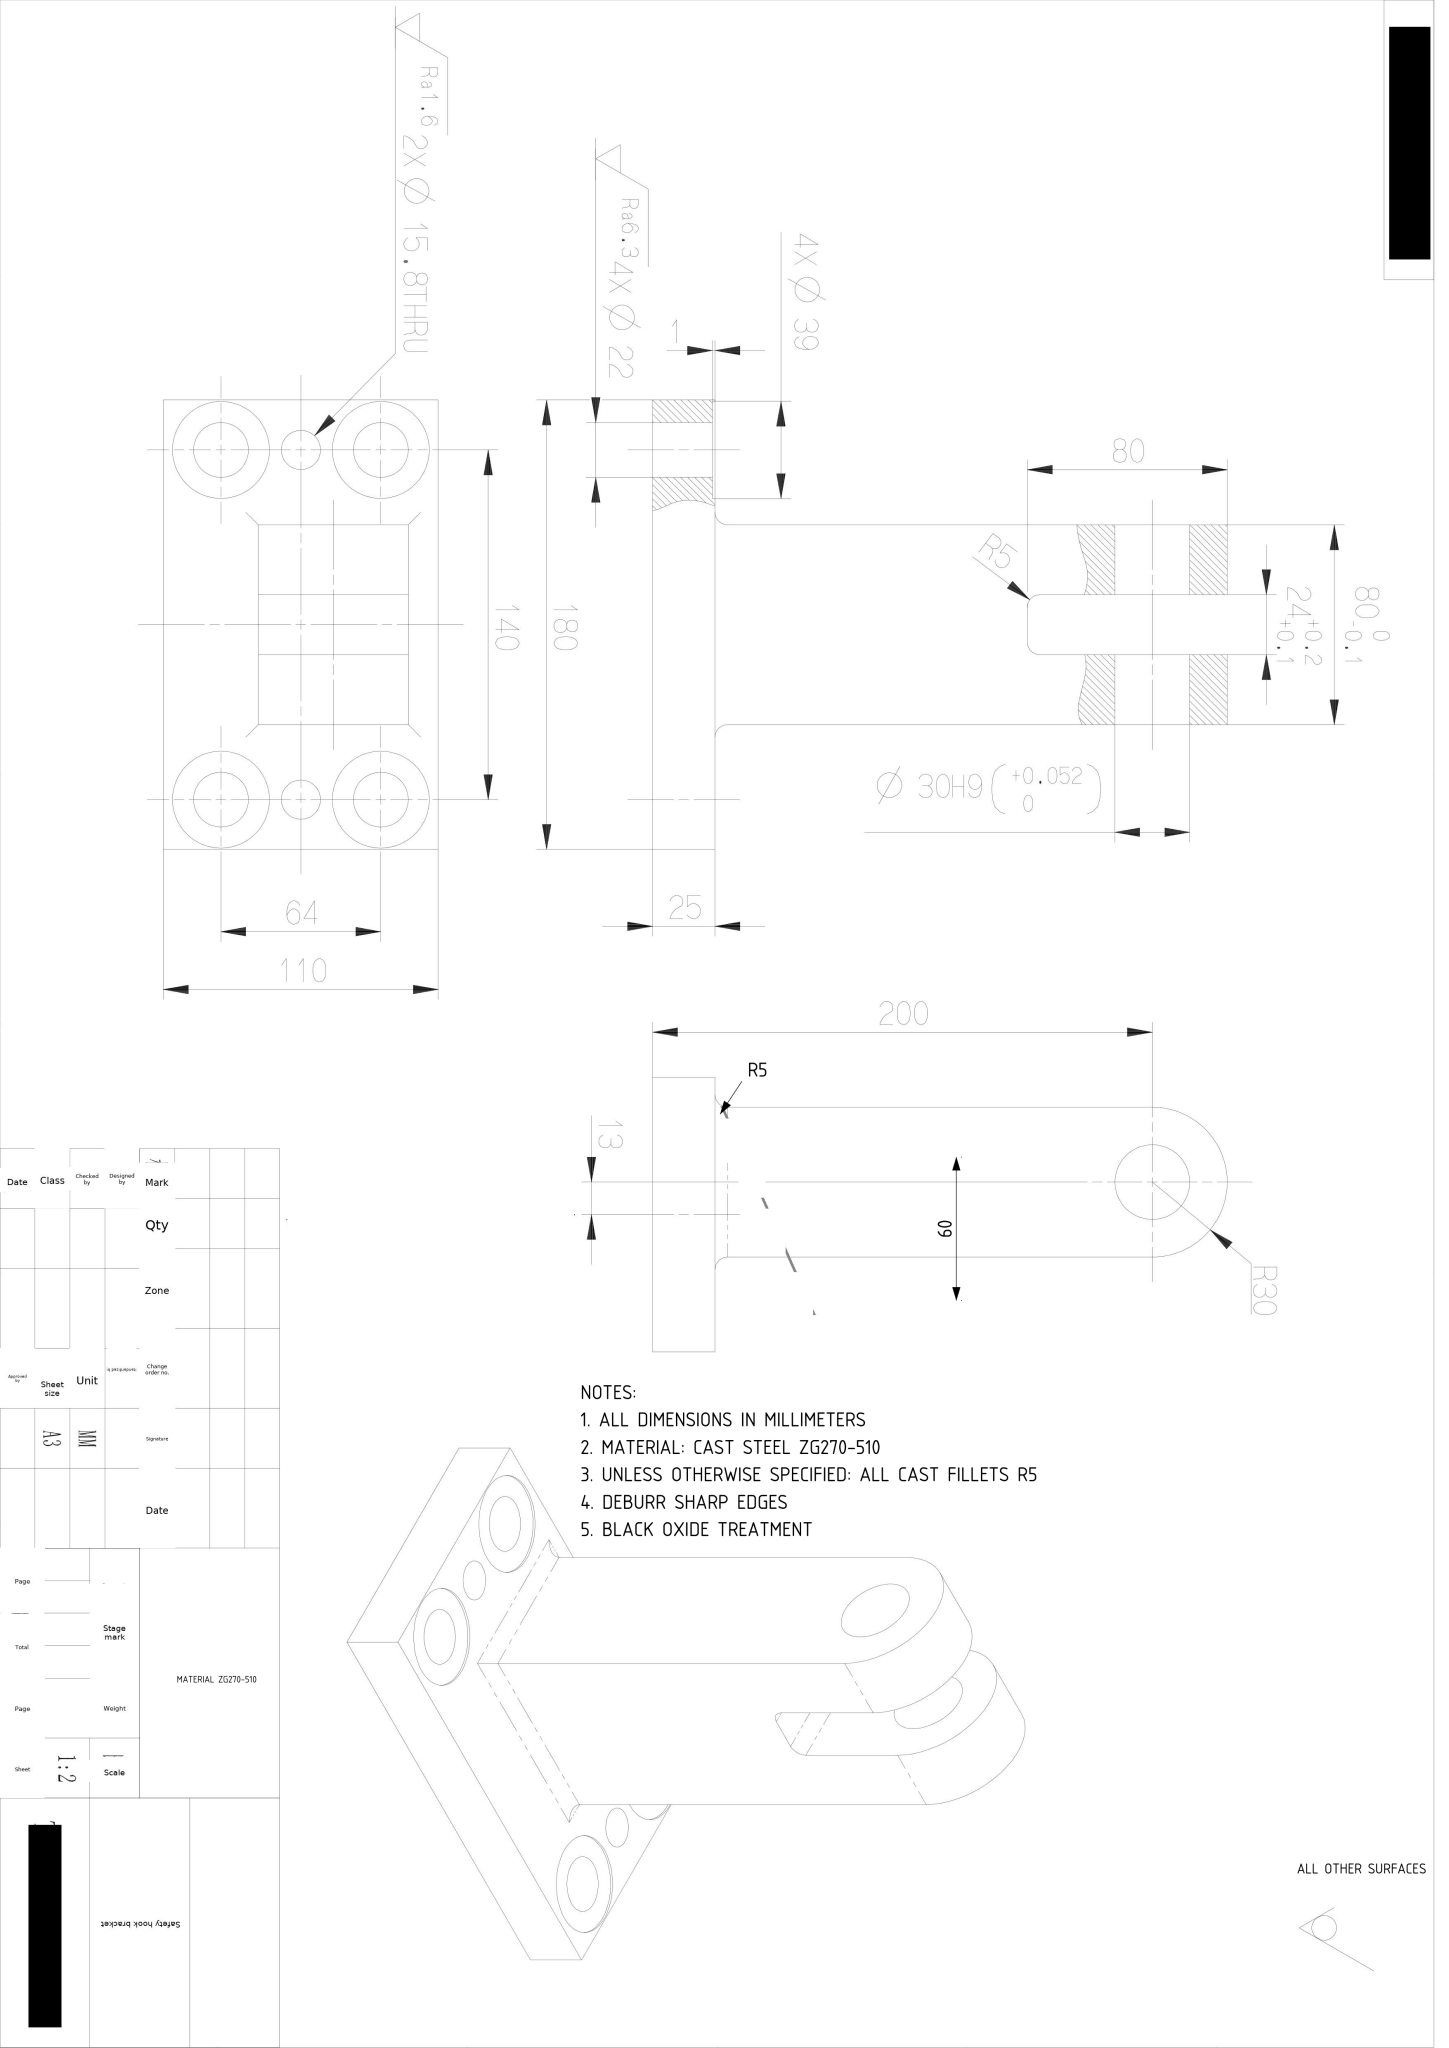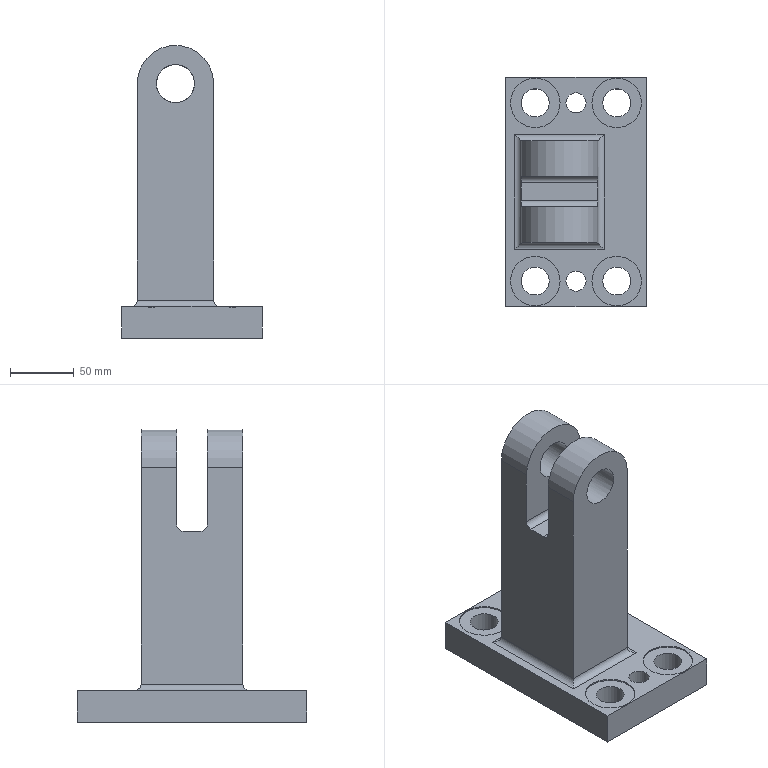Part | NX | mm | 1 solid | 37 faces | box 110 x 180 x 230 mm | volume 1253704 mm3 | cylinder 20 | plane 17 | commonest cylinder face diameters 10 x6 22 x4 39 x4 60 x2 30 x2 15.8 x2
STEP:
#1=CARTESIAN_POINT('',(0.,0.,0.));
#2=DIRECTION('',(0.,0.,1.));
#3=DIRECTION('',(1.,0.,0.));
#4=AXIS2_PLACEMENT_3D('',#1,#2,#3);
#5=(LENGTH_UNIT()NAMED_UNIT(*)SI_UNIT(.MILLI.,.METRE.));
#6=UNCERTAINTY_MEASURE_WITH_UNIT(LENGTH_MEASURE(0.00002),#5,'','');
#7=(NAMED_UNIT(*)PLANE_ANGLE_UNIT()SI_UNIT($,.RADIAN.));
#8=PLANE_ANGLE_MEASURE_WITH_UNIT(PLANE_ANGLE_MEASURE(0.01745),#7);
#9=DIMENSIONAL_EXPONENTS(0.,0.,0.,0.,0.,0.,0.);
#10=(CONVERSION_BASED_UNIT('',#8)NAMED_UNIT(#9)PLANE_ANGLE_UNIT());
#11=(NAMED_UNIT(*)SI_UNIT($,.STERADIAN.)SOLID_ANGLE_UNIT());
#12=(GEOMETRIC_REPRESENTATION_CONTEXT(3)GLOBAL_UNCERTAINTY_ASSIGNED_CONTEXT((#6))GLOBAL_UNIT_ASSIGNED_CONTEXT((#5,#10,#11))REPRESENTATION_CONTEXT('',''));
#13=SHAPE_REPRESENTATION('',(#4),#12);
#14=CARTESIAN_POINT('',(17.,-40.,200.));
#15=VERTEX_POINT('',#14);
#16=CARTESIAN_POINT('',(17.,-40.,30.));
#17=VERTEX_POINT('',#16);
#18=CARTESIAN_POINT('',(17.,-40.,230.));
#19=DIRECTION('',(0.,0.,-1.));
#20=VECTOR('',#19,1.);
#21=LINE('',#18,#20);
#22=EDGE_CURVE('',#15,#17,#21,.T.);
#23=ORIENTED_EDGE('',*,*,#22,.T.);
#24=CARTESIAN_POINT('',(17.,40.,30.));
#25=VERTEX_POINT('',#24);
#26=CARTESIAN_POINT('',(17.,-40.,30.));
#27=DIRECTION('',(-0.,1.,0.));
#28=VECTOR('',#27,1.);
#29=LINE('',#26,#28);
#30=EDGE_CURVE('',#17,#25,#29,.T.);
#31=ORIENTED_EDGE('',*,*,#30,.T.);
#32=CARTESIAN_POINT('',(17.,40.,200.));
#33=VERTEX_POINT('',#32);
#34=CARTESIAN_POINT('',(17.,40.,230.));
#35=DIRECTION('',(0.,0.,-1.));
#36=VECTOR('',#35,1.);
#37=LINE('',#34,#36);
#38=EDGE_CURVE('',#33,#25,#37,.T.);
#39=ORIENTED_EDGE('',*,*,#38,.F.);
#40=CARTESIAN_POINT('',(17.,12.,200.));
#41=VERTEX_POINT('',#40);
#42=CARTESIAN_POINT('',(17.,12.,200.));
#43=DIRECTION('',(0.,-1.,0.));
#44=VECTOR('',#43,1.);
#45=LINE('',#42,#44);
#46=EDGE_CURVE('',#33,#41,#45,.T.);
#47=ORIENTED_EDGE('',*,*,#46,.T.);
#48=CARTESIAN_POINT('',(17.,12.,155.));
#49=VERTEX_POINT('',#48);
#50=CARTESIAN_POINT('',(17.,12.,150.));
#51=DIRECTION('',(0.,0.,1.));
#52=VECTOR('',#51,1.);
#53=LINE('',#50,#52);
#54=EDGE_CURVE('',#49,#41,#53,.T.);
#55=ORIENTED_EDGE('',*,*,#54,.F.);
#56=CARTESIAN_POINT('',(17.,7.,150.));
#57=VERTEX_POINT('',#56);
#58=CARTESIAN_POINT('',(17.,7.,155.));
#59=DIRECTION('',(-1.,-0.,0.));
#60=DIRECTION('',(0.,-1.,0.));
#61=AXIS2_PLACEMENT_3D('',#58,#59,#60);
#62=CIRCLE('',#61,5.);
#63=EDGE_CURVE('',#49,#57,#62,.T.);
#64=ORIENTED_EDGE('',*,*,#63,.T.);
#65=CARTESIAN_POINT('',(17.,-7.,150.));
#66=VERTEX_POINT('',#65);
#67=CARTESIAN_POINT('',(17.,-12.,150.));
#68=DIRECTION('',(0.,1.,0.));
#69=VECTOR('',#68,1.);
#70=LINE('',#67,#69);
#71=EDGE_CURVE('',#66,#57,#70,.T.);
#72=ORIENTED_EDGE('',*,*,#71,.F.);
#73=CARTESIAN_POINT('',(17.,-12.,155.));
#74=VERTEX_POINT('',#73);
#75=CARTESIAN_POINT('',(17.,-7.,155.));
#76=DIRECTION('',(-1.,-0.,0.));
#77=DIRECTION('',(0.,-1.,0.));
#78=AXIS2_PLACEMENT_3D('',#75,#76,#77);
#79=CIRCLE('',#78,5.);
#80=EDGE_CURVE('',#66,#74,#79,.T.);
#81=ORIENTED_EDGE('',*,*,#80,.T.);
#82=CARTESIAN_POINT('',(17.,-12.,200.));
#83=VERTEX_POINT('',#82);
#84=CARTESIAN_POINT('',(17.,-12.,255.));
#85=DIRECTION('',(0.,0.,-1.));
#86=VECTOR('',#85,1.);
#87=LINE('',#84,#86);
#88=EDGE_CURVE('',#83,#74,#87,.T.);
#89=ORIENTED_EDGE('',*,*,#88,.F.);
#90=CARTESIAN_POINT('',(17.,-40.,200.));
#91=DIRECTION('',(0.,-1.,0.));
#92=VECTOR('',#91,1.);
#93=LINE('',#90,#92);
#94=EDGE_CURVE('',#83,#15,#93,.T.);
#95=ORIENTED_EDGE('',*,*,#94,.T.);
#96=EDGE_LOOP('',(#23,#31,#39,#47,#55,#64,#72,#81,#89,#95));
#97=FACE_OUTER_BOUND('',#96,.T.);
#98=CARTESIAN_POINT('',(17.,-40.,230.));
#99=DIRECTION('',(-1.,-0.,0.));
#100=DIRECTION('',(0.,-1.,0.));
#101=AXIS2_PLACEMENT_3D('',#98,#99,#100);
#102=PLANE('',#101);
#103=ADVANCED_FACE('',(#97),#102,.F.);
#104=CARTESIAN_POINT('',(-55.,90.,0.));
#105=VERTEX_POINT('',#104);
#106=CARTESIAN_POINT('',(-55.,-90.,0.));
#107=VERTEX_POINT('',#106);
#108=CARTESIAN_POINT('',(-55.,90.,0.));
#109=DIRECTION('',(0.,-1.,0.));
#110=VECTOR('',#109,1.);
#111=LINE('',#108,#110);
#112=EDGE_CURVE('',#105,#107,#111,.T.);
#113=ORIENTED_EDGE('',*,*,#112,.T.);
#114=CARTESIAN_POINT('',(-55.,-90.,25.));
#115=VERTEX_POINT('',#114);
#116=CARTESIAN_POINT('',(-55.,-90.,25.));
#117=DIRECTION('',(0.,0.,-1.));
#118=VECTOR('',#117,1.);
#119=LINE('',#116,#118);
#120=EDGE_CURVE('',#115,#107,#119,.T.);
#121=ORIENTED_EDGE('',*,*,#120,.F.);
#122=CARTESIAN_POINT('',(-55.,90.,25.));
#123=VERTEX_POINT('',#122);
#124=CARTESIAN_POINT('',(-55.,90.,25.));
#125=DIRECTION('',(0.,-1.,0.));
#126=VECTOR('',#125,1.);
#127=LINE('',#124,#126);
#128=EDGE_CURVE('',#123,#115,#127,.T.);
#129=ORIENTED_EDGE('',*,*,#128,.F.);
#130=CARTESIAN_POINT('',(-55.,90.,25.));
#131=DIRECTION('',(0.,0.,-1.));
#132=VECTOR('',#131,1.);
#133=LINE('',#130,#132);
#134=EDGE_CURVE('',#123,#105,#133,.T.);
#135=ORIENTED_EDGE('',*,*,#134,.T.);
#136=EDGE_LOOP('',(#113,#121,#129,#135));
#137=FACE_OUTER_BOUND('',#136,.T.);
#138=CARTESIAN_POINT('',(-55.,90.,25.));
#139=DIRECTION('',(1.,0.,0.));
#140=DIRECTION('',(0.,0.,-1.));
#141=AXIS2_PLACEMENT_3D('',#138,#139,#140);
#142=PLANE('',#141);
#143=ADVANCED_FACE('',(#137),#142,.F.);
#144=CARTESIAN_POINT('',(55.,-90.,0.));
#145=VERTEX_POINT('',#144);
#146=CARTESIAN_POINT('',(-55.,-90.,0.));
#147=DIRECTION('',(1.,0.,0.));
#148=VECTOR('',#147,1.);
#149=LINE('',#146,#148);
#150=EDGE_CURVE('',#107,#145,#149,.T.);
#151=ORIENTED_EDGE('',*,*,#150,.T.);
#152=CARTESIAN_POINT('',(55.,-90.,25.));
#153=VERTEX_POINT('',#152);
#154=CARTESIAN_POINT('',(55.,-90.,25.));
#155=DIRECTION('',(0.,0.,-1.));
#156=VECTOR('',#155,1.);
#157=LINE('',#154,#156);
#158=EDGE_CURVE('',#153,#145,#157,.T.);
#159=ORIENTED_EDGE('',*,*,#158,.F.);
#160=CARTESIAN_POINT('',(-55.,-90.,25.));
#161=DIRECTION('',(1.,0.,0.));
#162=VECTOR('',#161,1.);
#163=LINE('',#160,#162);
#164=EDGE_CURVE('',#115,#153,#163,.T.);
#165=ORIENTED_EDGE('',*,*,#164,.F.);
#166=ORIENTED_EDGE('',*,*,#120,.T.);
#167=EDGE_LOOP('',(#151,#159,#165,#166));
#168=FACE_OUTER_BOUND('',#167,.T.);
#169=CARTESIAN_POINT('',(-55.,-90.,25.));
#170=DIRECTION('',(-0.,1.,0.));
#171=DIRECTION('',(-1.,-0.,0.));
#172=AXIS2_PLACEMENT_3D('',#169,#170,#171);
#173=PLANE('',#172);
#174=ADVANCED_FACE('',(#168),#173,.F.);
#175=CARTESIAN_POINT('',(55.,90.,0.));
#176=VERTEX_POINT('',#175);
#177=CARTESIAN_POINT('',(55.,-90.,0.));
#178=DIRECTION('',(0.,1.,0.));
#179=VECTOR('',#178,1.);
#180=LINE('',#177,#179);
#181=EDGE_CURVE('',#145,#176,#180,.T.);
#182=ORIENTED_EDGE('',*,*,#181,.T.);
#183=CARTESIAN_POINT('',(55.,90.,25.));
#184=VERTEX_POINT('',#183);
#185=CARTESIAN_POINT('',(55.,90.,25.));
#186=DIRECTION('',(0.,0.,-1.));
#187=VECTOR('',#186,1.);
#188=LINE('',#185,#187);
#189=EDGE_CURVE('',#184,#176,#188,.T.);
#190=ORIENTED_EDGE('',*,*,#189,.F.);
#191=CARTESIAN_POINT('',(55.,-90.,25.));
#192=DIRECTION('',(0.,1.,0.));
#193=VECTOR('',#192,1.);
#194=LINE('',#191,#193);
#195=EDGE_CURVE('',#153,#184,#194,.T.);
#196=ORIENTED_EDGE('',*,*,#195,.F.);
#197=ORIENTED_EDGE('',*,*,#158,.T.);
#198=EDGE_LOOP('',(#182,#190,#196,#197));
#199=FACE_OUTER_BOUND('',#198,.T.);
#200=CARTESIAN_POINT('',(55.,-90.,25.));
#201=DIRECTION('',(-1.,0.,0.));
#202=DIRECTION('',(0.,0.,1.));
#203=AXIS2_PLACEMENT_3D('',#200,#201,#202);
#204=PLANE('',#203);
#205=ADVANCED_FACE('',(#199),#204,.F.);
#206=CARTESIAN_POINT('',(55.,90.,0.));
#207=DIRECTION('',(-1.,-0.,0.));
#208=VECTOR('',#207,1.);
#209=LINE('',#206,#208);
#210=EDGE_CURVE('',#176,#105,#209,.T.);
#211=ORIENTED_EDGE('',*,*,#210,.T.);
#212=ORIENTED_EDGE('',*,*,#134,.F.);
#213=CARTESIAN_POINT('',(55.,90.,25.));
#214=DIRECTION('',(-1.,-0.,0.));
#215=VECTOR('',#214,1.);
#216=LINE('',#213,#215);
#217=EDGE_CURVE('',#184,#123,#216,.T.);
#218=ORIENTED_EDGE('',*,*,#217,.F.);
#219=ORIENTED_EDGE('',*,*,#189,.T.);
#220=EDGE_LOOP('',(#211,#212,#218,#219));
#221=FACE_OUTER_BOUND('',#220,.T.);
#222=CARTESIAN_POINT('',(55.,90.,25.));
#223=DIRECTION('',(0.,-1.,0.));
#224=DIRECTION('',(1.,0.,0.));
#225=AXIS2_PLACEMENT_3D('',#222,#223,#224);
#226=PLANE('',#225);
#227=ADVANCED_FACE('',(#221),#226,.F.);
#228=CARTESIAN_POINT('',(22.,-45.,25.));
#229=VERTEX_POINT('',#228);
#230=CARTESIAN_POINT('',(-48.,-45.,25.));
#231=VERTEX_POINT('',#230);
#232=CARTESIAN_POINT('',(0.,-45.,25.));
#233=DIRECTION('',(-1.,-0.,0.));
#234=VECTOR('',#233,1.);
#235=LINE('',#232,#234);
#236=EDGE_CURVE('',#229,#231,#235,.T.);
#237=ORIENTED_EDGE('',*,*,#236,.T.);
#238=CARTESIAN_POINT('',(-48.,45.,25.));
#239=VERTEX_POINT('',#238);
#240=CARTESIAN_POINT('',(-48.,-0.,25.));
#241=DIRECTION('',(-0.,1.,0.));
#242=VECTOR('',#241,1.);
#243=LINE('',#240,#242);
#244=EDGE_CURVE('',#231,#239,#243,.T.);
#245=ORIENTED_EDGE('',*,*,#244,.T.);
#246=CARTESIAN_POINT('',(22.,45.,25.));
#247=VERTEX_POINT('',#246);
#248=CARTESIAN_POINT('',(-0.,45.,25.));
#249=DIRECTION('',(1.,0.,0.));
#250=VECTOR('',#249,1.);
#251=LINE('',#248,#250);
#252=EDGE_CURVE('',#239,#247,#251,.T.);
#253=ORIENTED_EDGE('',*,*,#252,.T.);
#254=CARTESIAN_POINT('',(22.,0.,25.));
#255=DIRECTION('',(0.,-1.,0.));
#256=VECTOR('',#255,1.);
#257=LINE('',#254,#256);
#258=EDGE_CURVE('',#247,#229,#257,.T.);
#259=ORIENTED_EDGE('',*,*,#258,.T.);
#260=EDGE_LOOP('',(#237,#245,#253,#259));
#261=FACE_BOUND('',#260,.T.);
#262=CARTESIAN_POINT('',(-7.9,70.,25.));
#263=VERTEX_POINT('',#262);
#264=CARTESIAN_POINT('',(0.,70.,25.));
#265=DIRECTION('',(0.,0.,-1.));
#266=DIRECTION('',(-1.,0.,0.));
#267=AXIS2_PLACEMENT_3D('',#264,#265,#266);
#268=CIRCLE('',#267,7.9);
#269=EDGE_CURVE('',#263,#263,#268,.T.);
#270=ORIENTED_EDGE('',*,*,#269,.T.);
#271=EDGE_LOOP('',(#270));
#272=FACE_BOUND('',#271,.T.);
#273=CARTESIAN_POINT('',(-7.9,-70.,25.));
#274=VERTEX_POINT('',#273);
#275=CARTESIAN_POINT('',(0.,-70.,25.));
#276=DIRECTION('',(0.,0.,-1.));
#277=DIRECTION('',(-1.,0.,0.));
#278=AXIS2_PLACEMENT_3D('',#275,#276,#277);
#279=CIRCLE('',#278,7.9);
#280=EDGE_CURVE('',#274,#274,#279,.T.);
#281=ORIENTED_EDGE('',*,*,#280,.T.);
#282=EDGE_LOOP('',(#281));
#283=FACE_BOUND('',#282,.T.);
#284=CARTESIAN_POINT('',(12.5,70.,25.));
#285=VERTEX_POINT('',#284);
#286=CARTESIAN_POINT('',(32.,70.,25.));
#287=DIRECTION('',(0.,0.,-1.));
#288=DIRECTION('',(-1.,0.,0.));
#289=AXIS2_PLACEMENT_3D('',#286,#287,#288);
#290=CIRCLE('',#289,19.5);
#291=EDGE_CURVE('',#285,#285,#290,.T.);
#292=ORIENTED_EDGE('',*,*,#291,.T.);
#293=EDGE_LOOP('',(#292));
#294=FACE_BOUND('',#293,.T.);
#295=CARTESIAN_POINT('',(12.5,-70.,25.));
#296=VERTEX_POINT('',#295);
#297=CARTESIAN_POINT('',(32.,-70.,25.));
#298=DIRECTION('',(0.,0.,-1.));
#299=DIRECTION('',(-1.,0.,0.));
#300=AXIS2_PLACEMENT_3D('',#297,#298,#299);
#301=CIRCLE('',#300,19.5);
#302=EDGE_CURVE('',#296,#296,#301,.T.);
#303=ORIENTED_EDGE('',*,*,#302,.T.);
#304=EDGE_LOOP('',(#303));
#305=FACE_BOUND('',#304,.T.);
#306=CARTESIAN_POINT('',(-51.5,70.,25.));
#307=VERTEX_POINT('',#306);
#308=CARTESIAN_POINT('',(-32.,70.,25.));
#309=DIRECTION('',(0.,0.,-1.));
#310=DIRECTION('',(-1.,0.,0.));
#311=AXIS2_PLACEMENT_3D('',#308,#309,#310);
#312=CIRCLE('',#311,19.5);
#313=EDGE_CURVE('',#307,#307,#312,.T.);
#314=ORIENTED_EDGE('',*,*,#313,.T.);
#315=EDGE_LOOP('',(#314));
#316=FACE_BOUND('',#315,.T.);
#317=CARTESIAN_POINT('',(-51.5,-70.,25.));
#318=VERTEX_POINT('',#317);
#319=CARTESIAN_POINT('',(-32.,-70.,25.));
#320=DIRECTION('',(0.,0.,-1.));
#321=DIRECTION('',(-1.,0.,0.));
#322=AXIS2_PLACEMENT_3D('',#319,#320,#321);
#323=CIRCLE('',#322,19.5);
#324=EDGE_CURVE('',#318,#318,#323,.T.);
#325=ORIENTED_EDGE('',*,*,#324,.T.);
#326=EDGE_LOOP('',(#325));
#327=FACE_BOUND('',#326,.T.);
#328=ORIENTED_EDGE('',*,*,#128,.T.);
#329=ORIENTED_EDGE('',*,*,#164,.T.);
#330=ORIENTED_EDGE('',*,*,#195,.T.);
#331=ORIENTED_EDGE('',*,*,#217,.T.);
#332=EDGE_LOOP('',(#328,#329,#330,#331));
#333=FACE_BOUND('',#332,.T.);
#334=CARTESIAN_POINT('',(0.,0.,25.));
#335=DIRECTION('',(0.,0.,1.));
#336=DIRECTION('',(1.,0.,0.));
#337=AXIS2_PLACEMENT_3D('',#334,#335,#336);
#338=PLANE('',#337);
#339=ADVANCED_FACE('',(#261,#272,#283,#294,#305,#316,#327,#333),#338,.T.);
#340=CARTESIAN_POINT('',(7.9,70.,0.));
#341=VERTEX_POINT('',#340);
#342=CARTESIAN_POINT('',(0.,70.,0.));
#343=DIRECTION('',(0.,0.,1.));
#344=DIRECTION('',(1.,0.,0.));
#345=AXIS2_PLACEMENT_3D('',#342,#343,#344);
#346=CIRCLE('',#345,7.9);
#347=EDGE_CURVE('',#341,#341,#346,.T.);
#348=ORIENTED_EDGE('',*,*,#347,.T.);
#349=EDGE_LOOP('',(#348));
#350=FACE_BOUND('',#349,.T.);
#351=CARTESIAN_POINT('',(7.9,-70.,0.));
#352=VERTEX_POINT('',#351);
#353=CARTESIAN_POINT('',(0.,-70.,0.));
#354=DIRECTION('',(0.,0.,1.));
#355=DIRECTION('',(1.,0.,0.));
#356=AXIS2_PLACEMENT_3D('',#353,#354,#355);
#357=CIRCLE('',#356,7.9);
#358=EDGE_CURVE('',#352,#352,#357,.T.);
#359=ORIENTED_EDGE('',*,*,#358,.T.);
#360=EDGE_LOOP('',(#359));
#361=FACE_BOUND('',#360,.T.);
#362=CARTESIAN_POINT('',(43.,70.,0.));
#363=VERTEX_POINT('',#362);
#364=CARTESIAN_POINT('',(32.,70.,0.));
#365=DIRECTION('',(0.,0.,1.));
#366=DIRECTION('',(1.,0.,0.));
#367=AXIS2_PLACEMENT_3D('',#364,#365,#366);
#368=CIRCLE('',#367,11.);
#369=EDGE_CURVE('',#363,#363,#368,.T.);
#370=ORIENTED_EDGE('',*,*,#369,.T.);
#371=EDGE_LOOP('',(#370));
#372=FACE_BOUND('',#371,.T.);
#373=CARTESIAN_POINT('',(43.,-70.,0.));
#374=VERTEX_POINT('',#373);
#375=CARTESIAN_POINT('',(32.,-70.,0.));
#376=DIRECTION('',(0.,0.,1.));
#377=DIRECTION('',(1.,0.,0.));
#378=AXIS2_PLACEMENT_3D('',#375,#376,#377);
#379=CIRCLE('',#378,11.);
#380=EDGE_CURVE('',#374,#374,#379,.T.);
#381=ORIENTED_EDGE('',*,*,#380,.T.);
#382=EDGE_LOOP('',(#381));
#383=FACE_BOUND('',#382,.T.);
#384=CARTESIAN_POINT('',(-21.,70.,0.));
#385=VERTEX_POINT('',#384);
#386=CARTESIAN_POINT('',(-32.,70.,0.));
#387=DIRECTION('',(0.,0.,1.));
#388=DIRECTION('',(1.,0.,0.));
#389=AXIS2_PLACEMENT_3D('',#386,#387,#388);
#390=CIRCLE('',#389,11.);
#391=EDGE_CURVE('',#385,#385,#390,.T.);
#392=ORIENTED_EDGE('',*,*,#391,.T.);
#393=EDGE_LOOP('',(#392));
#394=FACE_BOUND('',#393,.T.);
#395=CARTESIAN_POINT('',(-21.,-70.,0.));
#396=VERTEX_POINT('',#395);
#397=CARTESIAN_POINT('',(-32.,-70.,0.));
#398=DIRECTION('',(0.,0.,1.));
#399=DIRECTION('',(1.,0.,0.));
#400=AXIS2_PLACEMENT_3D('',#397,#398,#399);
#401=CIRCLE('',#400,11.);
#402=EDGE_CURVE('',#396,#396,#401,.T.);
#403=ORIENTED_EDGE('',*,*,#402,.T.);
#404=EDGE_LOOP('',(#403));
#405=FACE_BOUND('',#404,.T.);
#406=ORIENTED_EDGE('',*,*,#112,.F.);
#407=ORIENTED_EDGE('',*,*,#210,.F.);
#408=ORIENTED_EDGE('',*,*,#181,.F.);
#409=ORIENTED_EDGE('',*,*,#150,.F.);
#410=EDGE_LOOP('',(#406,#407,#408,#409));
#411=FACE_BOUND('',#410,.T.);
#412=CARTESIAN_POINT('',(0.,0.,0.));
#413=DIRECTION('',(0.,0.,1.));
#414=DIRECTION('',(1.,0.,0.));
#415=AXIS2_PLACEMENT_3D('',#412,#413,#414);
#416=PLANE('',#415);
#417=ADVANCED_FACE('',(#350,#361,#372,#383,#394,#405,#411),#416,.F.);
#418=CARTESIAN_POINT('',(-43.,40.,200.));
#419=VERTEX_POINT('',#418);
#420=CARTESIAN_POINT('',(-43.,40.,30.));
#421=VERTEX_POINT('',#420);
#422=CARTESIAN_POINT('',(-43.,40.,230.));
#423=DIRECTION('',(0.,0.,-1.));
#424=VECTOR('',#423,1.);
#425=LINE('',#422,#424);
#426=EDGE_CURVE('',#419,#421,#425,.T.);
#427=ORIENTED_EDGE('',*,*,#426,.T.);
#428=CARTESIAN_POINT('',(-43.,-40.,30.));
#429=VERTEX_POINT('',#428);
#430=CARTESIAN_POINT('',(-43.,40.,30.));
#431=DIRECTION('',(0.,-1.,0.));
#432=VECTOR('',#431,1.);
#433=LINE('',#430,#432);
#434=EDGE_CURVE('',#421,#429,#433,.T.);
#435=ORIENTED_EDGE('',*,*,#434,.T.);
#436=CARTESIAN_POINT('',(-43.,-40.,200.));
#437=VERTEX_POINT('',#436);
#438=CARTESIAN_POINT('',(-43.,-40.,230.));
#439=DIRECTION('',(0.,0.,-1.));
#440=VECTOR('',#439,1.);
#441=LINE('',#438,#440);
#442=EDGE_CURVE('',#437,#429,#441,.T.);
#443=ORIENTED_EDGE('',*,*,#442,.F.);
#444=CARTESIAN_POINT('',(-43.,-12.,200.));
#445=VERTEX_POINT('',#444);
#446=CARTESIAN_POINT('',(-43.,-12.,200.));
#447=DIRECTION('',(-0.,1.,0.));
#448=VECTOR('',#447,1.);
#449=LINE('',#446,#448);
#450=EDGE_CURVE('',#437,#445,#449,.T.);
#451=ORIENTED_EDGE('',*,*,#450,.T.);
#452=CARTESIAN_POINT('',(-43.,-12.,155.));
#453=VERTEX_POINT('',#452);
#454=CARTESIAN_POINT('',(-43.,-12.,230.));
#455=DIRECTION('',(-0.,0.,-1.));
#456=VECTOR('',#455,1.);
#457=LINE('',#454,#456);
#458=EDGE_CURVE('',#445,#453,#457,.T.);
#459=ORIENTED_EDGE('',*,*,#458,.T.);
#460=CARTESIAN_POINT('',(-43.,-7.,150.));
#461=VERTEX_POINT('',#460);
#462=CARTESIAN_POINT('',(-43.,-7.,155.));
#463=DIRECTION('',(1.,0.,0.));
#464=DIRECTION('',(0.,1.,0.));
#465=AXIS2_PLACEMENT_3D('',#462,#463,#464);
#466=CIRCLE('',#465,5.);
#467=EDGE_CURVE('',#453,#461,#466,.T.);
#468=ORIENTED_EDGE('',*,*,#467,.T.);
#469=CARTESIAN_POINT('',(-43.,7.,150.));
#470=VERTEX_POINT('',#469);
#471=CARTESIAN_POINT('',(-43.,40.,150.));
#472=DIRECTION('',(-0.,1.,0.));
#473=VECTOR('',#472,1.);
#474=LINE('',#471,#473);
#475=EDGE_CURVE('',#461,#470,#474,.T.);
#476=ORIENTED_EDGE('',*,*,#475,.T.);
#477=CARTESIAN_POINT('',(-43.,12.,155.));
#478=VERTEX_POINT('',#477);
#479=CARTESIAN_POINT('',(-43.,7.,155.));
#480=DIRECTION('',(1.,0.,0.));
#481=DIRECTION('',(0.,1.,0.));
#482=AXIS2_PLACEMENT_3D('',#479,#480,#481);
#483=CIRCLE('',#482,5.);
#484=EDGE_CURVE('',#470,#478,#483,.T.);
#485=ORIENTED_EDGE('',*,*,#484,.T.);
#486=CARTESIAN_POINT('',(-43.,12.,200.));
#487=VERTEX_POINT('',#486);
#488=CARTESIAN_POINT('',(-43.,12.,230.));
#489=DIRECTION('',(-0.,0.,1.));
#490=VECTOR('',#489,1.);
#491=LINE('',#488,#490);
#492=EDGE_CURVE('',#478,#487,#491,.T.);
#493=ORIENTED_EDGE('',*,*,#492,.T.);
#494=CARTESIAN_POINT('',(-43.,40.,200.));
#495=DIRECTION('',(-0.,1.,0.));
#496=VECTOR('',#495,1.);
#497=LINE('',#494,#496);
#498=EDGE_CURVE('',#487,#419,#497,.T.);
#499=ORIENTED_EDGE('',*,*,#498,.T.);
#500=EDGE_LOOP('',(#427,#435,#443,#451,#459,#468,#476,#485,#493,#499));
#501=FACE_OUTER_BOUND('',#500,.T.);
#502=CARTESIAN_POINT('',(-43.,40.,230.));
#503=DIRECTION('',(1.,0.,0.));
#504=DIRECTION('',(-0.,1.,0.));
#505=AXIS2_PLACEMENT_3D('',#502,#503,#504);
#506=PLANE('',#505);
#507=ADVANCED_FACE('',(#501),#506,.F.);
#508=CARTESIAN_POINT('',(-28.,-40.,200.));
#509=VERTEX_POINT('',#508);
#510=CARTESIAN_POINT('',(-13.,-40.,200.));
#511=DIRECTION('',(-0.,1.,0.));
#512=DIRECTION('',(-1.,0.,0.));
#513=AXIS2_PLACEMENT_3D('',#510,#511,#512);
#514=CIRCLE('',#513,15.);
#515=EDGE_CURVE('',#509,#509,#514,.T.);
#516=ORIENTED_EDGE('',*,*,#515,.T.);
#517=EDGE_LOOP('',(#516));
#518=FACE_BOUND('',#517,.T.);
#519=ORIENTED_EDGE('',*,*,#442,.T.);
#520=CARTESIAN_POINT('',(-43.,-40.,30.));
#521=DIRECTION('',(1.,0.,0.));
#522=VECTOR('',#521,1.);
#523=LINE('',#520,#522);
#524=EDGE_CURVE('',#429,#17,#523,.T.);
#525=ORIENTED_EDGE('',*,*,#524,.T.);
#526=ORIENTED_EDGE('',*,*,#22,.F.);
#527=CARTESIAN_POINT('',(-13.,-40.,200.));
#528=DIRECTION('',(0.,-1.,0.));
#529=DIRECTION('',(-1.,-0.,0.));
#530=AXIS2_PLACEMENT_3D('',#527,#528,#529);
#531=CIRCLE('',#530,30.);
#532=EDGE_CURVE('',#15,#437,#531,.T.);
#533=ORIENTED_EDGE('',*,*,#532,.T.);
#534=EDGE_LOOP('',(#519,#525,#526,#533));
#535=FACE_BOUND('',#534,.T.);
#536=CARTESIAN_POINT('',(-43.,-40.,230.));
#537=DIRECTION('',(-0.,1.,0.));
#538=DIRECTION('',(-1.,-0.,0.));
#539=AXIS2_PLACEMENT_3D('',#536,#537,#538);
#540=PLANE('',#539);
#541=ADVANCED_FACE('',(#518,#535),#540,.F.);
#542=CARTESIAN_POINT('',(2.,40.,200.));
#543=VERTEX_POINT('',#542);
#544=CARTESIAN_POINT('',(-13.,40.,200.));
#545=DIRECTION('',(0.,-1.,0.));
#546=DIRECTION('',(1.,0.,0.));
#547=AXIS2_PLACEMENT_3D('',#544,#545,#546);
#548=CIRCLE('',#547,15.);
#549=EDGE_CURVE('',#543,#543,#548,.T.);
#550=ORIENTED_EDGE('',*,*,#549,.T.);
#551=EDGE_LOOP('',(#550));
#552=FACE_BOUND('',#551,.T.);
#553=ORIENTED_EDGE('',*,*,#38,.T.);
#554=CARTESIAN_POINT('',(17.,40.,30.));
#555=DIRECTION('',(-1.,-0.,0.));
#556=VECTOR('',#555,1.);
#557=LINE('',#554,#556);
#558=EDGE_CURVE('',#25,#421,#557,.T.);
#559=ORIENTED_EDGE('',*,*,#558,.T.);
#560=ORIENTED_EDGE('',*,*,#426,.F.);
#561=CARTESIAN_POINT('',(-13.,40.,200.));
#562=DIRECTION('',(-0.,1.,0.));
#563=DIRECTION('',(1.,0.,0.));
#564=AXIS2_PLACEMENT_3D('',#561,#562,#563);
#565=CIRCLE('',#564,30.);
#566=EDGE_CURVE('',#419,#33,#565,.T.);
#567=ORIENTED_EDGE('',*,*,#566,.T.);
#568=EDGE_LOOP('',(#553,#559,#560,#567));
#569=FACE_BOUND('',#568,.T.);
#570=CARTESIAN_POINT('',(17.,40.,230.));
#571=DIRECTION('',(0.,-1.,0.));
#572=DIRECTION('',(1.,0.,0.));
#573=AXIS2_PLACEMENT_3D('',#570,#571,#572);
#574=PLANE('',#573);
#575=ADVANCED_FACE('',(#552,#569),#574,.F.);
#576=ORIENTED_EDGE('',*,*,#71,.T.);
#577=CARTESIAN_POINT('',(-43.,7.,150.));
#578=DIRECTION('',(-1.,0.,0.));
#579=VECTOR('',#578,1.);
#580=LINE('',#577,#579);
#581=EDGE_CURVE('',#57,#470,#580,.T.);
#582=ORIENTED_EDGE('',*,*,#581,.T.);
#583=ORIENTED_EDGE('',*,*,#475,.F.);
#584=CARTESIAN_POINT('',(17.,-7.,150.));
#585=DIRECTION('',(1.,0.,0.));
#586=VECTOR('',#585,1.);
#587=LINE('',#584,#586);
#588=EDGE_CURVE('',#461,#66,#587,.T.);
#589=ORIENTED_EDGE('',*,*,#588,.T.);
#590=EDGE_LOOP('',(#576,#582,#583,#589));
#591=FACE_OUTER_BOUND('',#590,.T.);
#592=CARTESIAN_POINT('',(-188.,-12.,150.));
#593=DIRECTION('',(0.,0.,-1.));
#594=DIRECTION('',(-1.,0.,0.));
#595=AXIS2_PLACEMENT_3D('',#592,#593,#594);
#596=PLANE('',#595);
#597=ADVANCED_FACE('',(#591),#596,.F.);
#598=CARTESIAN_POINT('',(-13.,-12.,185.));
#599=VERTEX_POINT('',#598);
#600=CARTESIAN_POINT('',(-13.,-12.,200.));
#601=DIRECTION('',(0.,-1.,-0.));
#602=DIRECTION('',(0.,0.,-1.));
#603=AXIS2_PLACEMENT_3D('',#600,#601,#602);
#604=CIRCLE('',#603,15.);
#605=EDGE_CURVE('',#599,#599,#604,.T.);
#606=ORIENTED_EDGE('',*,*,#605,.T.);
#607=EDGE_LOOP('',(#606));
#608=FACE_BOUND('',#607,.T.);
#609=ORIENTED_EDGE('',*,*,#88,.T.);
#610=CARTESIAN_POINT('',(-43.,-12.,155.));
#611=DIRECTION('',(-1.,0.,0.));
#612=VECTOR('',#611,1.);
#613=LINE('',#610,#612);
#614=EDGE_CURVE('',#74,#453,#613,.T.);
#615=ORIENTED_EDGE('',*,*,#614,.T.);
#616=ORIENTED_EDGE('',*,*,#458,.F.);
#617=CARTESIAN_POINT('',(-13.,-12.,200.));
#618=DIRECTION('',(0.,1.,0.));
#619=DIRECTION('',(0.,0.,-1.));
#620=AXIS2_PLACEMENT_3D('',#617,#618,#619);
#621=CIRCLE('',#620,30.);
#622=EDGE_CURVE('',#445,#83,#621,.T.);
#623=ORIENTED_EDGE('',*,*,#622,.T.);
#624=EDGE_LOOP('',(#609,#615,#616,#623));
#625=FACE_BOUND('',#624,.T.);
#626=CARTESIAN_POINT('',(-188.,-12.,255.));
#627=DIRECTION('',(0.,-1.,-0.));
#628=DIRECTION('',(0.,0.,-1.));
#629=AXIS2_PLACEMENT_3D('',#626,#627,#628);
#630=PLANE('',#629);
#631=ADVANCED_FACE('',(#608,#625),#630,.F.);
#632=CARTESIAN_POINT('',(-13.,12.,215.));
#633=VERTEX_POINT('',#632);
#634=CARTESIAN_POINT('',(-13.,12.,200.));
#635=DIRECTION('',(0.,1.,-0.));
#636=DIRECTION('',(0.,0.,1.));
#637=AXIS2_PLACEMENT_3D('',#634,#635,#636);
#638=CIRCLE('',#637,15.);
#639=EDGE_CURVE('',#633,#633,#638,.T.);
#640=ORIENTED_EDGE('',*,*,#639,.T.);
#641=EDGE_LOOP('',(#640));
#642=FACE_BOUND('',#641,.T.);
#643=ORIENTED_EDGE('',*,*,#492,.F.);
#644=CARTESIAN_POINT('',(17.,12.,155.));
#645=DIRECTION('',(1.,0.,0.));
#646=VECTOR('',#645,1.);
#647=LINE('',#644,#646);
#648=EDGE_CURVE('',#478,#49,#647,.T.);
#649=ORIENTED_EDGE('',*,*,#648,.T.);
#650=ORIENTED_EDGE('',*,*,#54,.T.);
#651=CARTESIAN_POINT('',(-13.,12.,200.));
#652=DIRECTION('',(0.,-1.,0.));
#653=DIRECTION('',(0.,0.,1.));
#654=AXIS2_PLACEMENT_3D('',#651,#652,#653);
#655=CIRCLE('',#654,30.);
#656=EDGE_CURVE('',#41,#487,#655,.T.);
#657=ORIENTED_EDGE('',*,*,#656,.T.);
#658=EDGE_LOOP('',(#643,#649,#650,#657));
#659=FACE_BOUND('',#658,.T.);
#660=CARTESIAN_POINT('',(-188.,12.,150.));
#661=DIRECTION('',(0.,1.,-0.));
#662=DIRECTION('',(0.,0.,1.));
#663=AXIS2_PLACEMENT_3D('',#660,#661,#662);
#664=PLANE('',#663);
#665=ADVANCED_FACE('',(#642,#659),#664,.F.);
#666=ORIENTED_EDGE('',*,*,#94,.F.);
#667=ORIENTED_EDGE('',*,*,#622,.F.);
#668=ORIENTED_EDGE('',*,*,#450,.F.);
#669=ORIENTED_EDGE('',*,*,#532,.F.);
#670=EDGE_LOOP('',(#666,#667,#668,#669));
#671=FACE_OUTER_BOUND('',#670,.T.);
#672=CARTESIAN_POINT('',(-13.,-0.,200.));
#673=DIRECTION('',(0.,-1.,0.));
#674=DIRECTION('',(1.,0.,0.));
#675=AXIS2_PLACEMENT_3D('',#672,#673,#674);
#676=CYLINDRICAL_SURFACE('',#675,30.);
#677=ADVANCED_FACE('',(#671),#676,.T.);
#678=ORIENTED_EDGE('',*,*,#46,.F.);
#679=ORIENTED_EDGE('',*,*,#566,.F.);
#680=ORIENTED_EDGE('',*,*,#498,.F.);
#681=ORIENTED_EDGE('',*,*,#656,.F.);
#682=EDGE_LOOP('',(#678,#679,#680,#681));
#683=FACE_OUTER_BOUND('',#682,.T.);
#684=CARTESIAN_POINT('',(-13.,-0.,200.));
#685=DIRECTION('',(0.,-1.,0.));
#686=DIRECTION('',(1.,0.,0.));
#687=AXIS2_PLACEMENT_3D('',#684,#685,#686);
#688=CYLINDRICAL_SURFACE('',#687,30.);
#689=ADVANCED_FACE('',(#683),#688,.T.);
#690=ORIENTED_EDGE('',*,*,#639,.F.);
#691=EDGE_LOOP('',(#690));
#692=FACE_BOUND('',#691,.T.);
#693=ORIENTED_EDGE('',*,*,#549,.F.);
#694=EDGE_LOOP('',(#693));
#695=FACE_BOUND('',#694,.T.);
#696=CARTESIAN_POINT('',(-13.,-40.,200.));
#697=DIRECTION('',(-0.,1.,0.));
#698=DIRECTION('',(-1.,0.,0.));
#699=AXIS2_PLACEMENT_3D('',#696,#697,#698);
#700=CYLINDRICAL_SURFACE('',#699,15.);
#701=ADVANCED_FACE('',(#692,#695),#700,.F.);
#702=ORIENTED_EDGE('',*,*,#515,.F.);
#703=EDGE_LOOP('',(#702));
#704=FACE_BOUND('',#703,.T.);
#705=ORIENTED_EDGE('',*,*,#605,.F.);
#706=EDGE_LOOP('',(#705));
#707=FACE_BOUND('',#706,.T.);
#708=CARTESIAN_POINT('',(-13.,-40.,200.));
#709=DIRECTION('',(-0.,1.,0.));
#710=DIRECTION('',(-1.,0.,0.));
#711=AXIS2_PLACEMENT_3D('',#708,#709,#710);
#712=CYLINDRICAL_SURFACE('',#711,15.);
#713=ADVANCED_FACE('',(#704,#707),#712,.F.);
#714=CARTESIAN_POINT('',(-43.,-70.,24.));
#715=VERTEX_POINT('',#714);
#716=CARTESIAN_POINT('',(-32.,-70.,24.));
#717=DIRECTION('',(0.,0.,1.));
#718=DIRECTION('',(-1.,0.,0.));
#719=AXIS2_PLACEMENT_3D('',#716,#717,#718);
#720=CIRCLE('',#719,11.);
#721=EDGE_CURVE('',#715,#715,#720,.T.);
#722=ORIENTED_EDGE('',*,*,#721,.T.);
#723=EDGE_LOOP('',(#722));
#724=FACE_BOUND('',#723,.T.);
#725=ORIENTED_EDGE('',*,*,#402,.F.);
#726=EDGE_LOOP('',(#725));
#727=FACE_BOUND('',#726,.T.);
#728=CARTESIAN_POINT('',(-32.,-70.,-25.));
#729=DIRECTION('',(0.,0.,-1.));
#730=DIRECTION('',(-1.,0.,0.));
#731=AXIS2_PLACEMENT_3D('',#728,#729,#730);
#732=CYLINDRICAL_SURFACE('',#731,11.);
#733=ADVANCED_FACE('',(#724,#727),#732,.F.);
#734=ORIENTED_EDGE('',*,*,#721,.F.);
#735=EDGE_LOOP('',(#734));
#736=FACE_BOUND('',#735,.T.);
#737=CARTESIAN_POINT('',(-51.5,-70.,24.));
#738=VERTEX_POINT('',#737);
#739=CARTESIAN_POINT('',(-32.,-70.,24.));
#740=DIRECTION('',(0.,0.,1.));
#741=DIRECTION('',(-1.,0.,0.));
#742=AXIS2_PLACEMENT_3D('',#739,#740,#741);
#743=CIRCLE('',#742,19.5);
#744=EDGE_CURVE('',#738,#738,#743,.T.);
#745=ORIENTED_EDGE('',*,*,#744,.T.);
#746=EDGE_LOOP('',(#745));
#747=FACE_BOUND('',#746,.T.);
#748=CARTESIAN_POINT('',(-32.,-70.,24.));
#749=DIRECTION('',(0.,0.,-1.));
#750=DIRECTION('',(-1.,0.,0.));
#751=AXIS2_PLACEMENT_3D('',#748,#749,#750);
#752=PLANE('',#751);
#753=ADVANCED_FACE('',(#736,#747),#752,.F.);
#754=ORIENTED_EDGE('',*,*,#744,.F.);
#755=EDGE_LOOP('',(#754));
#756=FACE_BOUND('',#755,.T.);
#757=ORIENTED_EDGE('',*,*,#324,.F.);
#758=EDGE_LOOP('',(#757));
#759=FACE_BOUND('',#758,.T.);
#760=CARTESIAN_POINT('',(-32.,-70.,25.));
#761=DIRECTION('',(0.,0.,-1.));
#762=DIRECTION('',(-1.,0.,0.));
#763=AXIS2_PLACEMENT_3D('',#760,#761,#762);
#764=CYLINDRICAL_SURFACE('',#763,19.5);
#765=ADVANCED_FACE('',(#756,#759),#764,.F.);
#766=CARTESIAN_POINT('',(-43.,70.,24.));
#767=VERTEX_POINT('',#766);
#768=CARTESIAN_POINT('',(-32.,70.,24.));
#769=DIRECTION('',(0.,0.,1.));
#770=DIRECTION('',(-1.,0.,0.));
#771=AXIS2_PLACEMENT_3D('',#768,#769,#770);
#772=CIRCLE('',#771,11.);
#773=EDGE_CURVE('',#767,#767,#772,.T.);
#774=ORIENTED_EDGE('',*,*,#773,.T.);
#775=EDGE_LOOP('',(#774));
#776=FACE_BOUND('',#775,.T.);
#777=ORIENTED_EDGE('',*,*,#391,.F.);
#778=EDGE_LOOP('',(#777));
#779=FACE_BOUND('',#778,.T.);
#780=CARTESIAN_POINT('',(-32.,70.,-25.));
#781=DIRECTION('',(0.,0.,-1.));
#782=DIRECTION('',(-1.,0.,0.));
#783=AXIS2_PLACEMENT_3D('',#780,#781,#782);
#784=CYLINDRICAL_SURFACE('',#783,11.);
#785=ADVANCED_FACE('',(#776,#779),#784,.F.);
#786=ORIENTED_EDGE('',*,*,#773,.F.);
#787=EDGE_LOOP('',(#786));
#788=FACE_BOUND('',#787,.T.);
#789=CARTESIAN_POINT('',(-51.5,70.,24.));
#790=VERTEX_POINT('',#789);
#791=CARTESIAN_POINT('',(-32.,70.,24.));
#792=DIRECTION('',(0.,0.,1.));
#793=DIRECTION('',(-1.,0.,0.));
#794=AXIS2_PLACEMENT_3D('',#791,#792,#793);
#795=CIRCLE('',#794,19.5);
#796=EDGE_CURVE('',#790,#790,#795,.T.);
#797=ORIENTED_EDGE('',*,*,#796,.T.);
#798=EDGE_LOOP('',(#797));
#799=FACE_BOUND('',#798,.T.);
#800=CARTESIAN_POINT('',(-32.,70.,24.));
#801=DIRECTION('',(0.,0.,-1.));
#802=DIRECTION('',(-1.,0.,0.));
#803=AXIS2_PLACEMENT_3D('',#800,#801,#802);
#804=PLANE('',#803);
#805=ADVANCED_FACE('',(#788,#799),#804,.F.);
#806=ORIENTED_EDGE('',*,*,#796,.F.);
#807=EDGE_LOOP('',(#806));
#808=FACE_BOUND('',#807,.T.);
#809=ORIENTED_EDGE('',*,*,#313,.F.);
#810=EDGE_LOOP('',(#809));
#811=FACE_BOUND('',#810,.T.);
#812=CARTESIAN_POINT('',(-32.,70.,25.));
#813=DIRECTION('',(0.,0.,-1.));
#814=DIRECTION('',(-1.,0.,0.));
#815=AXIS2_PLACEMENT_3D('',#812,#813,#814);
#816=CYLINDRICAL_SURFACE('',#815,19.5);
#817=ADVANCED_FACE('',(#808,#811),#816,.F.);
#818=CARTESIAN_POINT('',(21.,-70.,24.));
#819=VERTEX_POINT('',#818);
#820=CARTESIAN_POINT('',(32.,-70.,24.));
#821=DIRECTION('',(0.,0.,1.));
#822=DIRECTION('',(-1.,0.,0.));
#823=AXIS2_PLACEMENT_3D('',#820,#821,#822);
#824=CIRCLE('',#823,11.);
#825=EDGE_CURVE('',#819,#819,#824,.T.);
#826=ORIENTED_EDGE('',*,*,#825,.T.);
#827=EDGE_LOOP('',(#826));
#828=FACE_BOUND('',#827,.T.);
#829=ORIENTED_EDGE('',*,*,#380,.F.);
#830=EDGE_LOOP('',(#829));
#831=FACE_BOUND('',#830,.T.);
#832=CARTESIAN_POINT('',(32.,-70.,-25.));
#833=DIRECTION('',(0.,0.,-1.));
#834=DIRECTION('',(-1.,0.,0.));
#835=AXIS2_PLACEMENT_3D('',#832,#833,#834);
#836=CYLINDRICAL_SURFACE('',#835,11.);
#837=ADVANCED_FACE('',(#828,#831),#836,.F.);
#838=ORIENTED_EDGE('',*,*,#825,.F.);
#839=EDGE_LOOP('',(#838));
#840=FACE_BOUND('',#839,.T.);
#841=CARTESIAN_POINT('',(12.5,-70.,24.));
#842=VERTEX_POINT('',#841);
#843=CARTESIAN_POINT('',(32.,-70.,24.));
#844=DIRECTION('',(0.,0.,1.));
#845=DIRECTION('',(-1.,0.,0.));
#846=AXIS2_PLACEMENT_3D('',#843,#844,#845);
#847=CIRCLE('',#846,19.5);
#848=EDGE_CURVE('',#842,#842,#847,.T.);
#849=ORIENTED_EDGE('',*,*,#848,.T.);
#850=EDGE_LOOP('',(#849));
#851=FACE_BOUND('',#850,.T.);
#852=CARTESIAN_POINT('',(32.,-70.,24.));
#853=DIRECTION('',(0.,0.,-1.));
#854=DIRECTION('',(-1.,0.,0.));
#855=AXIS2_PLACEMENT_3D('',#852,#853,#854);
#856=PLANE('',#855);
#857=ADVANCED_FACE('',(#840,#851),#856,.F.);
#858=ORIENTED_EDGE('',*,*,#848,.F.);
#859=EDGE_LOOP('',(#858));
#860=FACE_BOUND('',#859,.T.);
#861=ORIENTED_EDGE('',*,*,#302,.F.);
#862=EDGE_LOOP('',(#861));
#863=FACE_BOUND('',#862,.T.);
#864=CARTESIAN_POINT('',(32.,-70.,25.));
#865=DIRECTION('',(0.,0.,-1.));
#866=DIRECTION('',(-1.,0.,0.));
#867=AXIS2_PLACEMENT_3D('',#864,#865,#866);
#868=CYLINDRICAL_SURFACE('',#867,19.5);
#869=ADVANCED_FACE('',(#860,#863),#868,.F.);
#870=CARTESIAN_POINT('',(21.,70.,24.));
#871=VERTEX_POINT('',#870);
#872=CARTESIAN_POINT('',(32.,70.,24.));
#873=DIRECTION('',(0.,0.,1.));
#874=DIRECTION('',(-1.,0.,0.));
#875=AXIS2_PLACEMENT_3D('',#872,#873,#874);
#876=CIRCLE('',#875,11.);
#877=EDGE_CURVE('',#871,#871,#876,.T.);
#878=ORIENTED_EDGE('',*,*,#877,.T.);
#879=EDGE_LOOP('',(#878));
#880=FACE_BOUND('',#879,.T.);
#881=ORIENTED_EDGE('',*,*,#369,.F.);
#882=EDGE_LOOP('',(#881));
#883=FACE_BOUND('',#882,.T.);
#884=CARTESIAN_POINT('',(32.,70.,-25.));
#885=DIRECTION('',(0.,0.,-1.));
#886=DIRECTION('',(-1.,0.,0.));
#887=AXIS2_PLACEMENT_3D('',#884,#885,#886);
#888=CYLINDRICAL_SURFACE('',#887,11.);
#889=ADVANCED_FACE('',(#880,#883),#888,.F.);
#890=ORIENTED_EDGE('',*,*,#877,.F.);
#891=EDGE_LOOP('',(#890));
#892=FACE_BOUND('',#891,.T.);
#893=CARTESIAN_POINT('',(12.5,70.,24.));
#894=VERTEX_POINT('',#893);
#895=CARTESIAN_POINT('',(32.,70.,24.));
#896=DIRECTION('',(0.,0.,1.));
#897=DIRECTION('',(-1.,0.,0.));
#898=AXIS2_PLACEMENT_3D('',#895,#896,#897);
#899=CIRCLE('',#898,19.5);
#900=EDGE_CURVE('',#894,#894,#899,.T.);
#901=ORIENTED_EDGE('',*,*,#900,.T.);
#902=EDGE_LOOP('',(#901));
#903=FACE_BOUND('',#902,.T.);
#904=CARTESIAN_POINT('',(32.,70.,24.));
#905=DIRECTION('',(0.,0.,-1.));
#906=DIRECTION('',(-1.,0.,0.));
#907=AXIS2_PLACEMENT_3D('',#904,#905,#906);
#908=PLANE('',#907);
#909=ADVANCED_FACE('',(#892,#903),#908,.F.);
#910=ORIENTED_EDGE('',*,*,#900,.F.);
#911=EDGE_LOOP('',(#910));
#912=FACE_BOUND('',#911,.T.);
#913=ORIENTED_EDGE('',*,*,#291,.F.);
#914=EDGE_LOOP('',(#913));
#915=FACE_BOUND('',#914,.T.);
#916=CARTESIAN_POINT('',(32.,70.,25.));
#917=DIRECTION('',(0.,0.,-1.));
#918=DIRECTION('',(-1.,0.,0.));
#919=AXIS2_PLACEMENT_3D('',#916,#917,#918);
#920=CYLINDRICAL_SURFACE('',#919,19.5);
#921=ADVANCED_FACE('',(#912,#915),#920,.F.);
#922=ORIENTED_EDGE('',*,*,#280,.F.);
#923=EDGE_LOOP('',(#922));
#924=FACE_BOUND('',#923,.T.);
#925=ORIENTED_EDGE('',*,*,#358,.F.);
#926=EDGE_LOOP('',(#925));
#927=FACE_BOUND('',#926,.T.);
#928=CARTESIAN_POINT('',(0.,-70.,25.));
#929=DIRECTION('',(0.,0.,-1.));
#930=DIRECTION('',(-1.,0.,0.));
#931=AXIS2_PLACEMENT_3D('',#928,#929,#930);
#932=CYLINDRICAL_SURFACE('',#931,7.9);
#933=ADVANCED_FACE('',(#924,#927),#932,.F.);
#934=ORIENTED_EDGE('',*,*,#269,.F.);
#935=EDGE_LOOP('',(#934));
#936=FACE_BOUND('',#935,.T.);
#937=ORIENTED_EDGE('',*,*,#347,.F.);
#938=EDGE_LOOP('',(#937));
#939=FACE_BOUND('',#938,.T.);
#940=CARTESIAN_POINT('',(0.,70.,25.));
#941=DIRECTION('',(0.,0.,-1.));
#942=DIRECTION('',(-1.,0.,0.));
#943=AXIS2_PLACEMENT_3D('',#940,#941,#942);
#944=CYLINDRICAL_SURFACE('',#943,7.9);
#945=ADVANCED_FACE('',(#936,#939),#944,.F.);
#946=CARTESIAN_POINT('',(22.,-45.,30.));
#947=DIRECTION('',(0.7071,0.7071,0.));
#948=DIRECTION('',(-0.7071,0.7071,0.));
#949=AXIS2_PLACEMENT_3D('',#946,#947,#948);
#950=ELLIPSE('',#949,7.071,5.);
#951=EDGE_CURVE('',#229,#17,#950,.T.);
#952=ORIENTED_EDGE('',*,*,#951,.F.);
#953=ORIENTED_EDGE('',*,*,#258,.F.);
#954=CARTESIAN_POINT('',(22.,45.,30.));
#955=DIRECTION('',(0.7071,-0.7071,0.));
#956=DIRECTION('',(0.7071,0.7071,0.));
#957=AXIS2_PLACEMENT_3D('',#954,#955,#956);
#958=ELLIPSE('',#957,7.071,5.);
#959=EDGE_CURVE('',#25,#247,#958,.T.);
#960=ORIENTED_EDGE('',*,*,#959,.F.);
#961=ORIENTED_EDGE('',*,*,#30,.F.);
#962=EDGE_LOOP('',(#952,#953,#960,#961));
#963=FACE_OUTER_BOUND('',#962,.T.);
#964=CARTESIAN_POINT('',(22.,-40.,30.));
#965=DIRECTION('',(-0.,1.,0.));
#966=DIRECTION('',(-1.,0.,0.));
#967=AXIS2_PLACEMENT_3D('',#964,#965,#966);
#968=CYLINDRICAL_SURFACE('',#967,5.);
#969=ADVANCED_FACE('',(#963),#968,.F.);
#970=ORIENTED_EDGE('',*,*,#959,.T.);
#971=ORIENTED_EDGE('',*,*,#252,.F.);
#972=CARTESIAN_POINT('',(-48.,45.,30.));
#973=DIRECTION('',(0.7071,0.7071,0.));
#974=DIRECTION('',(-0.7071,0.7071,0.));
#975=AXIS2_PLACEMENT_3D('',#972,#973,#974);
#976=ELLIPSE('',#975,7.071,5.);
#977=EDGE_CURVE('',#421,#239,#976,.T.);
#978=ORIENTED_EDGE('',*,*,#977,.F.);
#979=ORIENTED_EDGE('',*,*,#558,.F.);
#980=EDGE_LOOP('',(#970,#971,#978,#979));
#981=FACE_OUTER_BOUND('',#980,.T.);
#982=CARTESIAN_POINT('',(17.,45.,30.));
#983=DIRECTION('',(-1.,-0.,0.));
#984=DIRECTION('',(0.,-1.,0.));
#985=AXIS2_PLACEMENT_3D('',#982,#983,#984);
#986=CYLINDRICAL_SURFACE('',#985,5.);
#987=ADVANCED_FACE('',(#981),#986,.F.);
#988=ORIENTED_EDGE('',*,*,#951,.T.);
#989=ORIENTED_EDGE('',*,*,#524,.F.);
#990=CARTESIAN_POINT('',(-48.,-45.,30.));
#991=DIRECTION('',(0.7071,-0.7071,0.));
#992=DIRECTION('',(0.7071,0.7071,0.));
#993=AXIS2_PLACEMENT_3D('',#990,#991,#992);
#994=ELLIPSE('',#993,7.071,5.);
#995=EDGE_CURVE('',#231,#429,#994,.T.);
#996=ORIENTED_EDGE('',*,*,#995,.F.);
#997=ORIENTED_EDGE('',*,*,#236,.F.);
#998=EDGE_LOOP('',(#988,#989,#996,#997));
#999=FACE_OUTER_BOUND('',#998,.T.);
#1000=CARTESIAN_POINT('',(-43.,-45.,30.));
#1001=DIRECTION('',(1.,0.,0.));
#1002=DIRECTION('',(0.,1.,0.));
#1003=AXIS2_PLACEMENT_3D('',#1000,#1001,#1002);
#1004=CYLINDRICAL_SURFACE('',#1003,5.);
#1005=ADVANCED_FACE('',(#999),#1004,.F.);
#1006=ORIENTED_EDGE('',*,*,#977,.T.);
#1007=ORIENTED_EDGE('',*,*,#244,.F.);
#1008=ORIENTED_EDGE('',*,*,#995,.T.);
#1009=ORIENTED_EDGE('',*,*,#434,.F.);
#1010=EDGE_LOOP('',(#1006,#1007,#1008,#1009));
#1011=FACE_OUTER_BOUND('',#1010,.T.);
#1012=CARTESIAN_POINT('',(-48.,40.,30.));
#1013=DIRECTION('',(0.,-1.,0.));
#1014=DIRECTION('',(1.,0.,0.));
#1015=AXIS2_PLACEMENT_3D('',#1012,#1013,#1014);
#1016=CYLINDRICAL_SURFACE('',#1015,5.);
#1017=ADVANCED_FACE('',(#1011),#1016,.F.);
#1018=ORIENTED_EDGE('',*,*,#63,.F.);
#1019=ORIENTED_EDGE('',*,*,#648,.F.);
#1020=ORIENTED_EDGE('',*,*,#484,.F.);
#1021=ORIENTED_EDGE('',*,*,#581,.F.);
#1022=EDGE_LOOP('',(#1018,#1019,#1020,#1021));
#1023=FACE_OUTER_BOUND('',#1022,.T.);
#1024=CARTESIAN_POINT('',(-188.,7.,155.));
#1025=DIRECTION('',(1.,0.,0.));
#1026=DIRECTION('',(0.,0.,-1.));
#1027=AXIS2_PLACEMENT_3D('',#1024,#1025,#1026);
#1028=CYLINDRICAL_SURFACE('',#1027,5.);
#1029=ADVANCED_FACE('',(#1023),#1028,.F.);
#1030=ORIENTED_EDGE('',*,*,#80,.F.);
#1031=ORIENTED_EDGE('',*,*,#588,.F.);
#1032=ORIENTED_EDGE('',*,*,#467,.F.);
#1033=ORIENTED_EDGE('',*,*,#614,.F.);
#1034=EDGE_LOOP('',(#1030,#1031,#1032,#1033));
#1035=FACE_OUTER_BOUND('',#1034,.T.);
#1036=CARTESIAN_POINT('',(-188.,-7.,155.));
#1037=DIRECTION('',(1.,0.,0.));
#1038=DIRECTION('',(0.,0.,-1.));
#1039=AXIS2_PLACEMENT_3D('',#1036,#1037,#1038);
#1040=CYLINDRICAL_SURFACE('',#1039,5.);
#1041=ADVANCED_FACE('',(#1035),#1040,.F.);
#1042=CLOSED_SHELL('',(#103,#143,#174,#205,#227,#339,#417,#507,#541,#575,#597,#631,#665,#677,#689,#701,#713,#733,#753,#765,#785,#805,#817,#837,#857,#869,#889,#909,#921,#933,#945,#969,#987,#1005,#1017,#1029,#1041));
#1043=MANIFOLD_SOLID_BREP('',#1042);
#1044=ADVANCED_BREP_SHAPE_REPRESENTATION('',(#1043),#12);
#1045=SHAPE_REPRESENTATION_RELATIONSHIP('','',#13,#1044);
#1046=PRESENTATION_LAYER_ASSIGNMENT('','',(#1043));
#1047=COLOUR_RGB('',0.5961,0.6667,0.6863);
#1048=FILL_AREA_STYLE_COLOUR('',#1047);
#1049=FILL_AREA_STYLE('',(#1048));
#1050=SURFACE_STYLE_FILL_AREA(#1049);
#1051=SURFACE_SIDE_STYLE('',(#1050));
#1052=SURFACE_STYLE_USAGE(.BOTH.,#1051);
#1053=PRESENTATION_STYLE_ASSIGNMENT((#1052));
#1054=STYLED_ITEM('',(#1053),#1043);
#1055=MECHANICAL_DESIGN_GEOMETRIC_PRESENTATION_REPRESENTATION('',(#1054),#12);